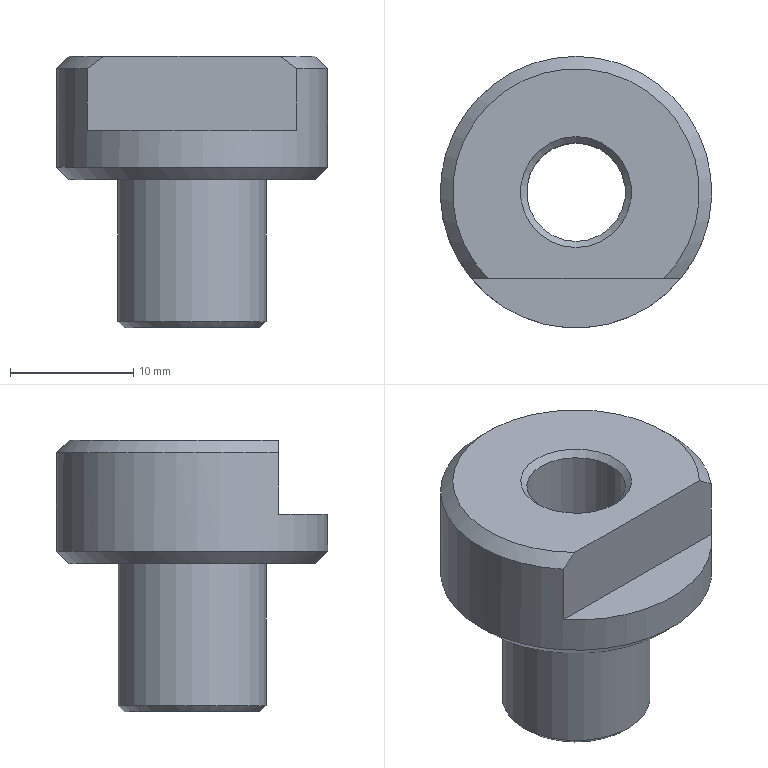Component | NX | DRILL_BUSH | 1 solid | 13 faces | box 22 x 22 x 22 mm | volume 3700 mm3 | plane 5 | cone 5 | cylinder 3 | commonest cylinder face diameters 12 x1 22 x1 8 x1
STEP:
#1=CARTESIAN_POINT('',(0.,0.,0.));
#2=DIRECTION('',(0.,0.,1.));
#3=DIRECTION('',(1.,0.,0.));
#4=AXIS2_PLACEMENT_3D('',#1,#2,#3);
#5=CARTESIAN_POINT('',(-15.,-13.5,92.));
#6=VERTEX_POINT('',#5);
#7=CARTESIAN_POINT('',(-15.,-18.,92.));
#8=DIRECTION('',(0.,0.,1.));
#9=DIRECTION('',(0.,1.,0.));
#10=AXIS2_PLACEMENT_3D('',#7,#8,#9);
#11=CIRCLE('',#10,4.5);
#12=CARTESIAN_POINT('',(-15.,-18.,92.));
#13=DIRECTION('',(0.,0.,-1.));
#14=DIRECTION('',(0.,1.,0.));
#15=AXIS2_PLACEMENT_3D('',#12,#13,#14);
#16=PLANE('',#15);
#17=CARTESIAN_POINT('',(4.5,0.));
#18=CARTESIAN_POINT('',(4.5,-7.794));
#19=CARTESIAN_POINT('',(-2.25,-3.897));
#20=CARTESIAN_POINT('',(-9.,-0.));
#21=CARTESIAN_POINT('',(-2.25,3.897));
#22=CARTESIAN_POINT('',(4.5,7.794));
#23=CARTESIAN_POINT('',(4.5,0.));
#24=(BOUNDED_CURVE()B_SPLINE_CURVE(2,(#17,#18,#19,#20,#21,#22,#23),.UNSPECIFIED.,.T.,.F.)B_SPLINE_CURVE_WITH_KNOTS((1,2,2,2,2,1),(-2.094,0.,2.094,4.189,6.283,8.378),.UNSPECIFIED.)CURVE()GEOMETRIC_REPRESENTATION_ITEM()RATIONAL_B_SPLINE_CURVE((1.,0.5,1.,0.5,1.,0.5,1.))REPRESENTATION_ITEM(''));
#25=(GEOMETRIC_REPRESENTATION_CONTEXT(2)PARAMETRIC_REPRESENTATION_CONTEXT()REPRESENTATION_CONTEXT('',''));
#26=DEFINITIONAL_REPRESENTATION('',(#24),#25);
#27=PCURVE('',#16,#26);
#28=CARTESIAN_POINT('',(-15.,-18.,92.5));
#29=DIRECTION('',(0.,0.,-1.));
#30=DIRECTION('',(0.,1.,0.));
#31=AXIS2_PLACEMENT_3D('',#28,#29,#30);
#32=CONICAL_SURFACE('',#31,4.,0.7854);
#33=CARTESIAN_POINT('',(6.283,0.5));
#34=DIRECTION('',(-1.,0.));
#35=VECTOR('',#34,1.);
#36=LINE('',#33,#35);
#37=(GEOMETRIC_REPRESENTATION_CONTEXT(2)PARAMETRIC_REPRESENTATION_CONTEXT()REPRESENTATION_CONTEXT('',''));
#38=DEFINITIONAL_REPRESENTATION('',(#36),#37);
#39=PCURVE('',#32,#38);
#40=SURFACE_CURVE('',#11,(#27,#39),.PCURVE_S1.);
#41=EDGE_CURVE('',#6,#6,#40,.T.);
#42=ORIENTED_EDGE('',*,*,#41,.T.);
#43=EDGE_LOOP('',(#42));
#44=FACE_BOUND('',#43,.T.);
#45=CARTESIAN_POINT('',(-15.,-12.5,92.));
#46=VERTEX_POINT('',#45);
#47=CARTESIAN_POINT('',(-15.,-18.,92.));
#48=DIRECTION('',(0.,0.,-1.));
#49=DIRECTION('',(0.,1.,0.));
#50=AXIS2_PLACEMENT_3D('',#47,#48,#49);
#51=CIRCLE('',#50,5.5);
#52=CARTESIAN_POINT('',(0.,0.));
#53=DIRECTION('',(1.,0.));
#54=AXIS2_PLACEMENT_2D('',#52,#53);
#55=CIRCLE('',#54,5.5);
#56=(GEOMETRIC_REPRESENTATION_CONTEXT(2)PARAMETRIC_REPRESENTATION_CONTEXT()REPRESENTATION_CONTEXT('',''));
#57=DEFINITIONAL_REPRESENTATION('',(#55),#56);
#58=PCURVE('',#16,#57);
#59=CARTESIAN_POINT('',(-15.,-18.,92.5));
#60=DIRECTION('',(0.,0.,1.));
#61=DIRECTION('',(0.,-1.,0.));
#62=AXIS2_PLACEMENT_3D('',#59,#60,#61);
#63=CONICAL_SURFACE('',#62,6.,0.7854);
#64=CARTESIAN_POINT('',(9.425,-0.5));
#65=DIRECTION('',(-1.,0.));
#66=VECTOR('',#65,1.);
#67=LINE('',#64,#66);
#68=(GEOMETRIC_REPRESENTATION_CONTEXT(2)PARAMETRIC_REPRESENTATION_CONTEXT()REPRESENTATION_CONTEXT('',''));
#69=DEFINITIONAL_REPRESENTATION('',(#67),#68);
#70=PCURVE('',#63,#69);
#71=SURFACE_CURVE('',#51,(#58,#70),.PCURVE_S1.);
#72=EDGE_CURVE('',#46,#46,#71,.T.);
#73=ORIENTED_EDGE('',*,*,#72,.T.);
#74=EDGE_LOOP('',(#73));
#75=FACE_BOUND('',#74,.T.);
#76=ADVANCED_FACE('',(#44,#75),#16,.T.);
#77=CARTESIAN_POINT('',(-15.,-12.,92.5));
#78=VERTEX_POINT('',#77);
#79=CARTESIAN_POINT('',(-15.,-18.,92.5));
#80=DIRECTION('',(0.,0.,1.));
#81=DIRECTION('',(0.,1.,0.));
#82=AXIS2_PLACEMENT_3D('',#79,#80,#81);
#83=CIRCLE('',#82,6.);
#84=CARTESIAN_POINT('',(-15.,-18.,92.));
#85=DIRECTION('',(0.,0.,1.));
#86=DIRECTION('',(0.,-1.,0.));
#87=AXIS2_PLACEMENT_3D('',#84,#85,#86);
#88=CYLINDRICAL_SURFACE('',#87,6.);
#89=CARTESIAN_POINT('',(3.142,0.5));
#90=DIRECTION('',(1.,0.));
#91=VECTOR('',#90,1.);
#92=LINE('',#89,#91);
#93=(GEOMETRIC_REPRESENTATION_CONTEXT(2)PARAMETRIC_REPRESENTATION_CONTEXT()REPRESENTATION_CONTEXT('',''));
#94=DEFINITIONAL_REPRESENTATION('',(#92),#93);
#95=PCURVE('',#88,#94);
#96=CARTESIAN_POINT('',(3.142,0.));
#97=DIRECTION('',(1.,0.));
#98=VECTOR('',#97,1.);
#99=LINE('',#96,#98);
#100=(GEOMETRIC_REPRESENTATION_CONTEXT(2)PARAMETRIC_REPRESENTATION_CONTEXT()REPRESENTATION_CONTEXT('',''));
#101=DEFINITIONAL_REPRESENTATION('',(#99),#100);
#102=PCURVE('',#63,#101);
#103=SURFACE_CURVE('',#83,(#95,#102),.PCURVE_S1.);
#104=EDGE_CURVE('',#78,#78,#103,.T.);
#105=ORIENTED_EDGE('',*,*,#104,.T.);
#106=CARTESIAN_POINT('',(-15.,-12.,104.));
#107=VERTEX_POINT('',#106);
#108=CARTESIAN_POINT('',(-15.,-12.,92.5));
#109=CARTESIAN_POINT('',(-15.,-12.,104.));
#110=B_SPLINE_CURVE_WITH_KNOTS('',1,(#108,#109),.UNSPECIFIED.,.F.,.F.,(2,2),(0.5,12.),.PIECEWISE_BEZIER_KNOTS.);
#111=CARTESIAN_POINT('',(9.425,0.));
#112=DIRECTION('',(0.,1.));
#113=VECTOR('',#112,1.);
#114=LINE('',#111,#113);
#115=(GEOMETRIC_REPRESENTATION_CONTEXT(2)PARAMETRIC_REPRESENTATION_CONTEXT()REPRESENTATION_CONTEXT('',''));
#116=DEFINITIONAL_REPRESENTATION('',(#114),#115);
#117=PCURVE('',#88,#116);
#118=CARTESIAN_POINT('',(3.142,0.));
#119=DIRECTION('',(0.,1.));
#120=VECTOR('',#119,1.);
#121=LINE('',#118,#120);
#122=(GEOMETRIC_REPRESENTATION_CONTEXT(2)PARAMETRIC_REPRESENTATION_CONTEXT()REPRESENTATION_CONTEXT('',''));
#123=DEFINITIONAL_REPRESENTATION('',(#121),#122);
#124=PCURVE('',#88,#123);
#125=SEAM_CURVE('',#110,(#117,#124),.PCURVE_S1.);
#126=EDGE_CURVE('',#78,#107,#125,.T.);
#127=ORIENTED_EDGE('',*,*,#126,.T.);
#128=CARTESIAN_POINT('',(-15.,-18.,104.));
#129=DIRECTION('',(0.,0.,1.));
#130=DIRECTION('',(0.,1.,0.));
#131=AXIS2_PLACEMENT_3D('',#128,#129,#130);
#132=CIRCLE('',#131,6.);
#133=CARTESIAN_POINT('',(3.142,12.));
#134=DIRECTION('',(1.,0.));
#135=VECTOR('',#134,1.);
#136=LINE('',#133,#135);
#137=(GEOMETRIC_REPRESENTATION_CONTEXT(2)PARAMETRIC_REPRESENTATION_CONTEXT()REPRESENTATION_CONTEXT('',''));
#138=DEFINITIONAL_REPRESENTATION('',(#136),#137);
#139=PCURVE('',#88,#138);
#140=CARTESIAN_POINT('',(-15.,-18.,104.));
#141=DIRECTION('',(0.,0.,-1.));
#142=DIRECTION('',(0.,1.,0.));
#143=AXIS2_PLACEMENT_3D('',#140,#141,#142);
#144=PLANE('',#143);
#145=CARTESIAN_POINT('',(6.,0.));
#146=CARTESIAN_POINT('',(6.,-10.392));
#147=CARTESIAN_POINT('',(-3.,-5.196));
#148=CARTESIAN_POINT('',(-12.,-0.));
#149=CARTESIAN_POINT('',(-3.,5.196));
#150=CARTESIAN_POINT('',(6.,10.392));
#151=CARTESIAN_POINT('',(6.,0.));
#152=(BOUNDED_CURVE()B_SPLINE_CURVE(2,(#145,#146,#147,#148,#149,#150,#151),.UNSPECIFIED.,.T.,.F.)B_SPLINE_CURVE_WITH_KNOTS((1,2,2,2,2,1),(-2.094,0.,2.094,4.189,6.283,8.378),.UNSPECIFIED.)CURVE()GEOMETRIC_REPRESENTATION_ITEM()RATIONAL_B_SPLINE_CURVE((1.,0.5,1.,0.5,1.,0.5,1.))REPRESENTATION_ITEM(''));
#153=(GEOMETRIC_REPRESENTATION_CONTEXT(2)PARAMETRIC_REPRESENTATION_CONTEXT()REPRESENTATION_CONTEXT('',''));
#154=DEFINITIONAL_REPRESENTATION('',(#152),#153);
#155=PCURVE('',#144,#154);
#156=SURFACE_CURVE('',#132,(#139,#155),.PCURVE_S1.);
#157=EDGE_CURVE('',#107,#107,#156,.T.);
#158=ORIENTED_EDGE('',*,*,#157,.F.);
#159=ORIENTED_EDGE('',*,*,#126,.F.);
#160=EDGE_LOOP('',(#105,#127,#158,#159));
#161=FACE_BOUND('',#160,.T.);
#162=ADVANCED_FACE('',(#161),#88,.T.);
#163=CARTESIAN_POINT('',(-15.,-22.5,114.));
#164=VERTEX_POINT('',#163);
#165=CARTESIAN_POINT('',(-15.,-18.,114.));
#166=DIRECTION('',(0.,0.,-1.));
#167=DIRECTION('',(0.,-1.,0.));
#168=AXIS2_PLACEMENT_3D('',#165,#166,#167);
#169=CIRCLE('',#168,4.5);
#170=CARTESIAN_POINT('',(-15.,-18.,114.));
#171=DIRECTION('',(0.,0.,1.));
#172=DIRECTION('',(0.,-1.,0.));
#173=AXIS2_PLACEMENT_3D('',#170,#171,#172);
#174=PLANE('',#173);
#175=CARTESIAN_POINT('',(4.5,0.));
#176=CARTESIAN_POINT('',(4.5,-7.794));
#177=CARTESIAN_POINT('',(-2.25,-3.897));
#178=CARTESIAN_POINT('',(-9.,-0.));
#179=CARTESIAN_POINT('',(-2.25,3.897));
#180=CARTESIAN_POINT('',(4.5,7.794));
#181=CARTESIAN_POINT('',(4.5,0.));
#182=(BOUNDED_CURVE()B_SPLINE_CURVE(2,(#175,#176,#177,#178,#179,#180,#181),.UNSPECIFIED.,.T.,.F.)B_SPLINE_CURVE_WITH_KNOTS((1,2,2,2,2,1),(-2.094,0.,2.094,4.189,6.283,8.378),.UNSPECIFIED.)CURVE()GEOMETRIC_REPRESENTATION_ITEM()RATIONAL_B_SPLINE_CURVE((1.,0.5,1.,0.5,1.,0.5,1.))REPRESENTATION_ITEM(''));
#183=(GEOMETRIC_REPRESENTATION_CONTEXT(2)PARAMETRIC_REPRESENTATION_CONTEXT()REPRESENTATION_CONTEXT('',''));
#184=DEFINITIONAL_REPRESENTATION('',(#182),#183);
#185=PCURVE('',#174,#184);
#186=CARTESIAN_POINT('',(-15.,-18.,114.));
#187=DIRECTION('',(0.,0.,1.));
#188=DIRECTION('',(0.,-1.,0.));
#189=AXIS2_PLACEMENT_3D('',#186,#187,#188);
#190=CONICAL_SURFACE('',#189,4.5,0.7854);
#191=CARTESIAN_POINT('',(6.283,0.));
#192=DIRECTION('',(-1.,0.));
#193=VECTOR('',#192,1.);
#194=LINE('',#191,#193);
#195=(GEOMETRIC_REPRESENTATION_CONTEXT(2)PARAMETRIC_REPRESENTATION_CONTEXT()REPRESENTATION_CONTEXT('',''));
#196=DEFINITIONAL_REPRESENTATION('',(#194),#195);
#197=PCURVE('',#190,#196);
#198=SURFACE_CURVE('',#169,(#185,#197),.PCURVE_S1.);
#199=EDGE_CURVE('',#164,#164,#198,.T.);
#200=ORIENTED_EDGE('',*,*,#199,.T.);
#201=EDGE_LOOP('',(#200));
#202=FACE_BOUND('',#201,.T.);
#203=CARTESIAN_POINT('',(-7.859,-25.,114.));
#204=VERTEX_POINT('',#203);
#205=CARTESIAN_POINT('',(-22.141,-25.,114.));
#206=VERTEX_POINT('',#205);
#207=CARTESIAN_POINT('',(-2.,-25.,114.));
#208=DIRECTION('',(-1.,-0.,0.));
#209=VECTOR('',#208,1.);
#210=LINE('',#207,#209);
#211=CARTESIAN_POINT('',(7.,13.));
#212=DIRECTION('',(0.,-1.));
#213=VECTOR('',#212,1.);
#214=LINE('',#211,#213);
#215=(GEOMETRIC_REPRESENTATION_CONTEXT(2)PARAMETRIC_REPRESENTATION_CONTEXT()REPRESENTATION_CONTEXT('',''));
#216=DEFINITIONAL_REPRESENTATION('',(#214),#215);
#217=PCURVE('',#174,#216);
#218=CARTESIAN_POINT('',(-2.,-25.,108.));
#219=DIRECTION('',(-0.,1.,0.));
#220=DIRECTION('',(-1.,-0.,0.));
#221=AXIS2_PLACEMENT_3D('',#218,#219,#220);
#222=PLANE('',#221);
#223=CARTESIAN_POINT('',(0.,6.));
#224=DIRECTION('',(1.,0.));
#225=VECTOR('',#224,1.);
#226=LINE('',#223,#225);
#227=(GEOMETRIC_REPRESENTATION_CONTEXT(2)PARAMETRIC_REPRESENTATION_CONTEXT()REPRESENTATION_CONTEXT('',''));
#228=DEFINITIONAL_REPRESENTATION('',(#226),#227);
#229=PCURVE('',#222,#228);
#230=SURFACE_CURVE('',#210,(#217,#229),.PCURVE_S1.);
#231=EDGE_CURVE('',#204,#206,#230,.T.);
#232=ORIENTED_EDGE('',*,*,#231,.F.);
#233=CARTESIAN_POINT('',(-15.,-18.,114.));
#234=DIRECTION('',(0.,0.,1.));
#235=DIRECTION('',(0.,-1.,0.));
#236=AXIS2_PLACEMENT_3D('',#233,#234,#235);
#237=CIRCLE('',#236,10.);
#238=CARTESIAN_POINT('',(0.,0.));
#239=DIRECTION('',(1.,0.));
#240=AXIS2_PLACEMENT_2D('',#238,#239);
#241=CIRCLE('',#240,10.);
#242=(GEOMETRIC_REPRESENTATION_CONTEXT(2)PARAMETRIC_REPRESENTATION_CONTEXT()REPRESENTATION_CONTEXT('',''));
#243=DEFINITIONAL_REPRESENTATION('',(#241),#242);
#244=PCURVE('',#174,#243);
#245=CARTESIAN_POINT('',(-15.,-18.,113.));
#246=DIRECTION('',(0.,0.,-1.));
#247=DIRECTION('',(0.,1.,0.));
#248=AXIS2_PLACEMENT_3D('',#245,#246,#247);
#249=CONICAL_SURFACE('',#248,11.,0.7854);
#250=CARTESIAN_POINT('',(3.142,-1.));
#251=DIRECTION('',(-1.,0.));
#252=VECTOR('',#251,1.);
#253=LINE('',#250,#252);
#254=(GEOMETRIC_REPRESENTATION_CONTEXT(2)PARAMETRIC_REPRESENTATION_CONTEXT()REPRESENTATION_CONTEXT('',''));
#255=DEFINITIONAL_REPRESENTATION('',(#253),#254);
#256=PCURVE('',#249,#255);
#257=SURFACE_CURVE('',#237,(#244,#256),.PCURVE_S1.);
#258=EDGE_CURVE('',#204,#206,#257,.T.);
#259=ORIENTED_EDGE('',*,*,#258,.T.);
#260=EDGE_LOOP('',(#232,#259));
#261=FACE_BOUND('',#260,.T.);
#262=ADVANCED_FACE('',(#202,#261),#174,.T.);
#263=CARTESIAN_POINT('',(-15.,-8.,104.));
#264=VERTEX_POINT('',#263);
#265=CARTESIAN_POINT('',(-15.,-18.,104.));
#266=DIRECTION('',(0.,0.,-1.));
#267=DIRECTION('',(0.,1.,0.));
#268=AXIS2_PLACEMENT_3D('',#265,#266,#267);
#269=CIRCLE('',#268,10.);
#270=CARTESIAN_POINT('',(0.,0.));
#271=DIRECTION('',(1.,0.));
#272=AXIS2_PLACEMENT_2D('',#270,#271);
#273=CIRCLE('',#272,10.);
#274=(GEOMETRIC_REPRESENTATION_CONTEXT(2)PARAMETRIC_REPRESENTATION_CONTEXT()REPRESENTATION_CONTEXT('',''));
#275=DEFINITIONAL_REPRESENTATION('',(#273),#274);
#276=PCURVE('',#144,#275);
#277=CARTESIAN_POINT('',(-15.,-18.,105.));
#278=DIRECTION('',(0.,0.,1.));
#279=DIRECTION('',(0.,-1.,0.));
#280=AXIS2_PLACEMENT_3D('',#277,#278,#279);
#281=CONICAL_SURFACE('',#280,11.,0.7854);
#282=CARTESIAN_POINT('',(9.425,-1.));
#283=DIRECTION('',(-1.,0.));
#284=VECTOR('',#283,1.);
#285=LINE('',#282,#284);
#286=(GEOMETRIC_REPRESENTATION_CONTEXT(2)PARAMETRIC_REPRESENTATION_CONTEXT()REPRESENTATION_CONTEXT('',''));
#287=DEFINITIONAL_REPRESENTATION('',(#285),#286);
#288=PCURVE('',#281,#287);
#289=SURFACE_CURVE('',#269,(#276,#288),.PCURVE_S1.);
#290=EDGE_CURVE('',#264,#264,#289,.T.);
#291=ORIENTED_EDGE('',*,*,#290,.T.);
#292=EDGE_LOOP('',(#291));
#293=FACE_BOUND('',#292,.T.);
#294=ORIENTED_EDGE('',*,*,#157,.T.);
#295=EDGE_LOOP('',(#294));
#296=FACE_BOUND('',#295,.T.);
#297=ADVANCED_FACE('',(#293,#296),#144,.T.);
#298=CARTESIAN_POINT('',(-15.,-7.,105.));
#299=VERTEX_POINT('',#298);
#300=CARTESIAN_POINT('',(-6.515,-25.,105.));
#301=VERTEX_POINT('',#300);
#302=CARTESIAN_POINT('',(-15.,-18.,105.));
#303=DIRECTION('',(0.,0.,1.));
#304=DIRECTION('',(0.,1.,0.));
#305=AXIS2_PLACEMENT_3D('',#302,#303,#304);
#306=CIRCLE('',#305,11.);
#307=CARTESIAN_POINT('',(-15.,-18.,104.));
#308=DIRECTION('',(0.,0.,1.));
#309=DIRECTION('',(0.,-1.,0.));
#310=AXIS2_PLACEMENT_3D('',#307,#308,#309);
#311=CYLINDRICAL_SURFACE('',#310,11.);
#312=CARTESIAN_POINT('',(3.142,1.));
#313=DIRECTION('',(1.,0.));
#314=VECTOR('',#313,1.);
#315=LINE('',#312,#314);
#316=(GEOMETRIC_REPRESENTATION_CONTEXT(2)PARAMETRIC_REPRESENTATION_CONTEXT()REPRESENTATION_CONTEXT('',''));
#317=DEFINITIONAL_REPRESENTATION('',(#315),#316);
#318=PCURVE('',#311,#317);
#319=CARTESIAN_POINT('',(3.142,0.));
#320=DIRECTION('',(1.,0.));
#321=VECTOR('',#320,1.);
#322=LINE('',#319,#321);
#323=(GEOMETRIC_REPRESENTATION_CONTEXT(2)PARAMETRIC_REPRESENTATION_CONTEXT()REPRESENTATION_CONTEXT('',''));
#324=DEFINITIONAL_REPRESENTATION('',(#322),#323);
#325=PCURVE('',#281,#324);
#326=SURFACE_CURVE('',#306,(#318,#325),.PCURVE_S1.);
#327=EDGE_CURVE('',#299,#301,#326,.T.);
#328=ORIENTED_EDGE('',*,*,#327,.T.);
#329=CARTESIAN_POINT('',(-6.515,-25.,108.));
#330=VERTEX_POINT('',#329);
#331=CARTESIAN_POINT('',(-6.515,-25.,105.));
#332=CARTESIAN_POINT('',(-6.515,-25.,108.));
#333=B_SPLINE_CURVE_WITH_KNOTS('',1,(#331,#332),.UNSPECIFIED.,.F.,.F.,(2,2),(1.,4.),.PIECEWISE_BEZIER_KNOTS.);
#334=CARTESIAN_POINT('',(7.164,0.));
#335=DIRECTION('',(0.,1.));
#336=VECTOR('',#335,1.);
#337=LINE('',#334,#336);
#338=(GEOMETRIC_REPRESENTATION_CONTEXT(2)PARAMETRIC_REPRESENTATION_CONTEXT()REPRESENTATION_CONTEXT('',''));
#339=DEFINITIONAL_REPRESENTATION('',(#337),#338);
#340=PCURVE('',#311,#339);
#341=CARTESIAN_POINT('',(0.881,0.));
#342=DIRECTION('',(0.,1.));
#343=VECTOR('',#342,1.);
#344=LINE('',#341,#343);
#345=(GEOMETRIC_REPRESENTATION_CONTEXT(2)PARAMETRIC_REPRESENTATION_CONTEXT()REPRESENTATION_CONTEXT('',''));
#346=DEFINITIONAL_REPRESENTATION('',(#344),#345);
#347=PCURVE('',#311,#346);
#348=SEAM_CURVE('',#333,(#340,#347),.PCURVE_S1.);
#349=EDGE_CURVE('',#301,#330,#348,.T.);
#350=ORIENTED_EDGE('',*,*,#349,.T.);
#351=CARTESIAN_POINT('',(-23.485,-25.,108.));
#352=VERTEX_POINT('',#351);
#353=CARTESIAN_POINT('',(-15.,-18.,108.));
#354=DIRECTION('',(0.,0.,-1.));
#355=DIRECTION('',(0.,-1.,0.));
#356=AXIS2_PLACEMENT_3D('',#353,#354,#355);
#357=CIRCLE('',#356,11.);
#358=CARTESIAN_POINT('',(12.566,4.));
#359=DIRECTION('',(-1.,0.));
#360=VECTOR('',#359,1.);
#361=LINE('',#358,#360);
#362=(GEOMETRIC_REPRESENTATION_CONTEXT(2)PARAMETRIC_REPRESENTATION_CONTEXT()REPRESENTATION_CONTEXT('',''));
#363=DEFINITIONAL_REPRESENTATION('',(#361),#362);
#364=PCURVE('',#311,#363);
#365=CARTESIAN_POINT('',(-15.,-18.,108.));
#366=DIRECTION('',(0.,0.,1.));
#367=DIRECTION('',(0.,-1.,0.));
#368=AXIS2_PLACEMENT_3D('',#365,#366,#367);
#369=PLANE('',#368);
#370=CARTESIAN_POINT('',(11.,0.));
#371=CARTESIAN_POINT('',(11.,-19.053));
#372=CARTESIAN_POINT('',(-5.5,-9.526));
#373=CARTESIAN_POINT('',(-22.,-0.));
#374=CARTESIAN_POINT('',(-5.5,9.526));
#375=CARTESIAN_POINT('',(11.,19.053));
#376=CARTESIAN_POINT('',(11.,0.));
#377=(BOUNDED_CURVE()B_SPLINE_CURVE(2,(#370,#371,#372,#373,#374,#375,#376),.UNSPECIFIED.,.T.,.F.)B_SPLINE_CURVE_WITH_KNOTS((1,2,2,2,2,1),(-2.094,0.,2.094,4.189,6.283,8.378),.UNSPECIFIED.)CURVE()GEOMETRIC_REPRESENTATION_ITEM()RATIONAL_B_SPLINE_CURVE((1.,0.5,1.,0.5,1.,0.5,1.))REPRESENTATION_ITEM(''));
#378=(GEOMETRIC_REPRESENTATION_CONTEXT(2)PARAMETRIC_REPRESENTATION_CONTEXT()REPRESENTATION_CONTEXT('',''));
#379=DEFINITIONAL_REPRESENTATION('',(#377),#378);
#380=PCURVE('',#369,#379);
#381=SURFACE_CURVE('',#357,(#364,#380),.PCURVE_S1.);
#382=EDGE_CURVE('',#330,#352,#381,.T.);
#383=ORIENTED_EDGE('',*,*,#382,.T.);
#384=CARTESIAN_POINT('',(-23.485,-25.,113.));
#385=VERTEX_POINT('',#384);
#386=CARTESIAN_POINT('',(-23.485,-25.,104.));
#387=DIRECTION('',(0.,0.,-1.));
#388=VECTOR('',#387,1.);
#389=LINE('',#386,#388);
#390=CARTESIAN_POINT('',(5.402,0.));
#391=DIRECTION('',(0.,-1.));
#392=VECTOR('',#391,1.);
#393=LINE('',#390,#392);
#394=(GEOMETRIC_REPRESENTATION_CONTEXT(2)PARAMETRIC_REPRESENTATION_CONTEXT()REPRESENTATION_CONTEXT('',''));
#395=DEFINITIONAL_REPRESENTATION('',(#393),#394);
#396=PCURVE('',#311,#395);
#397=CARTESIAN_POINT('',(21.485,-4.));
#398=DIRECTION('',(0.,-1.));
#399=VECTOR('',#398,1.);
#400=LINE('',#397,#399);
#401=(GEOMETRIC_REPRESENTATION_CONTEXT(2)PARAMETRIC_REPRESENTATION_CONTEXT()REPRESENTATION_CONTEXT('',''));
#402=DEFINITIONAL_REPRESENTATION('',(#400),#401);
#403=PCURVE('',#222,#402);
#404=SURFACE_CURVE('',#389,(#396,#403),.PCURVE_S1.);
#405=EDGE_CURVE('',#385,#352,#404,.T.);
#406=ORIENTED_EDGE('',*,*,#405,.F.);
#407=CARTESIAN_POINT('',(-6.515,-25.,113.));
#408=VERTEX_POINT('',#407);
#409=CARTESIAN_POINT('',(-15.,-18.,113.));
#410=DIRECTION('',(0.,0.,-1.));
#411=DIRECTION('',(0.,-1.,0.));
#412=AXIS2_PLACEMENT_3D('',#409,#410,#411);
#413=CIRCLE('',#412,11.);
#414=CARTESIAN_POINT('',(6.283,9.));
#415=DIRECTION('',(-1.,0.));
#416=VECTOR('',#415,1.);
#417=LINE('',#414,#416);
#418=(GEOMETRIC_REPRESENTATION_CONTEXT(2)PARAMETRIC_REPRESENTATION_CONTEXT()REPRESENTATION_CONTEXT('',''));
#419=DEFINITIONAL_REPRESENTATION('',(#417),#418);
#420=PCURVE('',#311,#419);
#421=CARTESIAN_POINT('',(-3.142,0.));
#422=DIRECTION('',(1.,0.));
#423=VECTOR('',#422,1.);
#424=LINE('',#421,#423);
#425=(GEOMETRIC_REPRESENTATION_CONTEXT(2)PARAMETRIC_REPRESENTATION_CONTEXT()REPRESENTATION_CONTEXT('',''));
#426=DEFINITIONAL_REPRESENTATION('',(#424),#425);
#427=PCURVE('',#249,#426);
#428=SURFACE_CURVE('',#413,(#420,#427),.PCURVE_S1.);
#429=EDGE_CURVE('',#385,#408,#428,.T.);
#430=ORIENTED_EDGE('',*,*,#429,.T.);
#431=CARTESIAN_POINT('',(-6.515,-25.,104.));
#432=DIRECTION('',(0.,0.,1.));
#433=VECTOR('',#432,1.);
#434=LINE('',#431,#433);
#435=CARTESIAN_POINT('',(0.881,0.));
#436=DIRECTION('',(0.,1.));
#437=VECTOR('',#436,1.);
#438=LINE('',#435,#437);
#439=(GEOMETRIC_REPRESENTATION_CONTEXT(2)PARAMETRIC_REPRESENTATION_CONTEXT()REPRESENTATION_CONTEXT('',''));
#440=DEFINITIONAL_REPRESENTATION('',(#438),#439);
#441=PCURVE('',#311,#440);
#442=CARTESIAN_POINT('',(4.515,-4.));
#443=DIRECTION('',(0.,1.));
#444=VECTOR('',#443,1.);
#445=LINE('',#442,#444);
#446=(GEOMETRIC_REPRESENTATION_CONTEXT(2)PARAMETRIC_REPRESENTATION_CONTEXT()REPRESENTATION_CONTEXT('',''));
#447=DEFINITIONAL_REPRESENTATION('',(#445),#446);
#448=PCURVE('',#222,#447);
#449=SURFACE_CURVE('',#434,(#441,#448),.PCURVE_S1.);
#450=EDGE_CURVE('',#330,#408,#449,.T.);
#451=ORIENTED_EDGE('',*,*,#450,.F.);
#452=ORIENTED_EDGE('',*,*,#349,.F.);
#453=CARTESIAN_POINT('',(-15.,-18.,105.));
#454=DIRECTION('',(0.,0.,1.));
#455=DIRECTION('',(0.,1.,0.));
#456=AXIS2_PLACEMENT_3D('',#453,#454,#455);
#457=CIRCLE('',#456,11.);
#458=CARTESIAN_POINT('',(-3.142,1.));
#459=DIRECTION('',(1.,0.));
#460=VECTOR('',#459,1.);
#461=LINE('',#458,#460);
#462=(GEOMETRIC_REPRESENTATION_CONTEXT(2)PARAMETRIC_REPRESENTATION_CONTEXT()REPRESENTATION_CONTEXT('',''));
#463=DEFINITIONAL_REPRESENTATION('',(#461),#462);
#464=PCURVE('',#311,#463);
#465=CARTESIAN_POINT('',(3.142,0.));
#466=DIRECTION('',(1.,0.));
#467=VECTOR('',#466,1.);
#468=LINE('',#465,#467);
#469=(GEOMETRIC_REPRESENTATION_CONTEXT(2)PARAMETRIC_REPRESENTATION_CONTEXT()REPRESENTATION_CONTEXT('',''));
#470=DEFINITIONAL_REPRESENTATION('',(#468),#469);
#471=PCURVE('',#281,#470);
#472=SURFACE_CURVE('',#457,(#464,#471),.PCURVE_S1.);
#473=EDGE_CURVE('',#301,#299,#472,.T.);
#474=ORIENTED_EDGE('',*,*,#473,.T.);
#475=EDGE_LOOP('',(#328,#350,#383,#406,#430,#451,#452,#474));
#476=FACE_BOUND('',#475,.T.);
#477=ADVANCED_FACE('',(#476),#311,.T.);
#478=ORIENTED_EDGE('',*,*,#450,.T.);
#479=CARTESIAN_POINT('',(-6.515,-25.,113.));
#480=CARTESIAN_POINT('',(-6.957,-25.,113.341));
#481=CARTESIAN_POINT('',(-7.404,-25.,113.676));
#482=CARTESIAN_POINT('',(-7.859,-25.,114.));
#483=B_SPLINE_CURVE_WITH_KNOTS('',3,(#479,#480,#481,#482),.UNSPECIFIED.,.F.,.F.,(4,4),(0.,1.),.PIECEWISE_BEZIER_KNOTS.);
#484=CARTESIAN_POINT('',(4.515,5.));
#485=CARTESIAN_POINT('',(4.957,5.341));
#486=CARTESIAN_POINT('',(5.404,5.676));
#487=CARTESIAN_POINT('',(5.859,6.));
#488=B_SPLINE_CURVE_WITH_KNOTS('',3,(#484,#485,#486,#487),.UNSPECIFIED.,.F.,.F.,(4,4),(0.,1.),.PIECEWISE_BEZIER_KNOTS.);
#489=(GEOMETRIC_REPRESENTATION_CONTEXT(2)PARAMETRIC_REPRESENTATION_CONTEXT()REPRESENTATION_CONTEXT('',''));
#490=DEFINITIONAL_REPRESENTATION('',(#488),#489);
#491=PCURVE('',#222,#490);
#492=CARTESIAN_POINT('',(2.261,-0.));
#493=CARTESIAN_POINT('',(2.346,-1.));
#494=B_SPLINE_CURVE_WITH_KNOTS('',1,(#492,#493),.UNSPECIFIED.,.F.,.F.,(2,2),(0.,1.),.PIECEWISE_BEZIER_KNOTS.);
#495=(GEOMETRIC_REPRESENTATION_CONTEXT(2)PARAMETRIC_REPRESENTATION_CONTEXT()REPRESENTATION_CONTEXT('',''));
#496=DEFINITIONAL_REPRESENTATION('',(#494),#495);
#497=PCURVE('',#249,#496);
#498=SURFACE_CURVE('',#483,(#491,#497),.PCURVE_S1.);
#499=EDGE_CURVE('',#408,#204,#498,.T.);
#500=ORIENTED_EDGE('',*,*,#499,.T.);
#501=ORIENTED_EDGE('',*,*,#231,.T.);
#502=CARTESIAN_POINT('',(-22.141,-25.,114.));
#503=CARTESIAN_POINT('',(-22.596,-25.,113.676));
#504=CARTESIAN_POINT('',(-23.043,-25.,113.341));
#505=CARTESIAN_POINT('',(-23.485,-25.,113.));
#506=B_SPLINE_CURVE_WITH_KNOTS('',3,(#502,#503,#504,#505),.UNSPECIFIED.,.F.,.F.,(4,4),(0.,1.),.PIECEWISE_BEZIER_KNOTS.);
#507=CARTESIAN_POINT('',(20.141,6.));
#508=CARTESIAN_POINT('',(20.596,5.676));
#509=CARTESIAN_POINT('',(21.043,5.341));
#510=CARTESIAN_POINT('',(21.485,5.));
#511=B_SPLINE_CURVE_WITH_KNOTS('',3,(#507,#508,#509,#510),.UNSPECIFIED.,.F.,.F.,(4,4),(0.,1.),.PIECEWISE_BEZIER_KNOTS.);
#512=(GEOMETRIC_REPRESENTATION_CONTEXT(2)PARAMETRIC_REPRESENTATION_CONTEXT()REPRESENTATION_CONTEXT('',''));
#513=DEFINITIONAL_REPRESENTATION('',(#511),#512);
#514=PCURVE('',#222,#513);
#515=CARTESIAN_POINT('',(-2.346,-1.));
#516=CARTESIAN_POINT('',(-2.261,0.));
#517=B_SPLINE_CURVE_WITH_KNOTS('',1,(#515,#516),.UNSPECIFIED.,.F.,.F.,(2,2),(0.,1.),.PIECEWISE_BEZIER_KNOTS.);
#518=(GEOMETRIC_REPRESENTATION_CONTEXT(2)PARAMETRIC_REPRESENTATION_CONTEXT()REPRESENTATION_CONTEXT('',''));
#519=DEFINITIONAL_REPRESENTATION('',(#517),#518);
#520=PCURVE('',#249,#519);
#521=SURFACE_CURVE('',#506,(#514,#520),.PCURVE_S1.);
#522=EDGE_CURVE('',#206,#385,#521,.T.);
#523=ORIENTED_EDGE('',*,*,#522,.T.);
#524=ORIENTED_EDGE('',*,*,#405,.T.);
#525=CARTESIAN_POINT('',(-2.,-25.,108.));
#526=DIRECTION('',(1.,0.,0.));
#527=VECTOR('',#526,1.);
#528=LINE('',#525,#527);
#529=CARTESIAN_POINT('',(0.,0.));
#530=DIRECTION('',(-1.,0.));
#531=VECTOR('',#530,1.);
#532=LINE('',#529,#531);
#533=(GEOMETRIC_REPRESENTATION_CONTEXT(2)PARAMETRIC_REPRESENTATION_CONTEXT()REPRESENTATION_CONTEXT('',''));
#534=DEFINITIONAL_REPRESENTATION('',(#532),#533);
#535=PCURVE('',#222,#534);
#536=CARTESIAN_POINT('',(7.,13.));
#537=DIRECTION('',(-0.,1.));
#538=VECTOR('',#537,1.);
#539=LINE('',#536,#538);
#540=(GEOMETRIC_REPRESENTATION_CONTEXT(2)PARAMETRIC_REPRESENTATION_CONTEXT()REPRESENTATION_CONTEXT('',''));
#541=DEFINITIONAL_REPRESENTATION('',(#539),#540);
#542=PCURVE('',#369,#541);
#543=SURFACE_CURVE('',#528,(#535,#542),.PCURVE_S1.);
#544=EDGE_CURVE('',#352,#330,#543,.T.);
#545=ORIENTED_EDGE('',*,*,#544,.T.);
#546=EDGE_LOOP('',(#478,#500,#501,#523,#524,#545));
#547=FACE_BOUND('',#546,.T.);
#548=ADVANCED_FACE('',(#547),#222,.F.);
#549=ORIENTED_EDGE('',*,*,#544,.F.);
#550=ORIENTED_EDGE('',*,*,#382,.F.);
#551=EDGE_LOOP('',(#549,#550));
#552=FACE_BOUND('',#551,.T.);
#553=ADVANCED_FACE('',(#552),#369,.T.);
#554=CARTESIAN_POINT('',(-15.,-14.,92.5));
#555=VERTEX_POINT('',#554);
#556=CARTESIAN_POINT('',(-15.,-18.,92.5));
#557=DIRECTION('',(0.,0.,-1.));
#558=DIRECTION('',(0.,1.,0.));
#559=AXIS2_PLACEMENT_3D('',#556,#557,#558);
#560=CIRCLE('',#559,4.);
#561=CARTESIAN_POINT('',(-15.,-18.,114.));
#562=DIRECTION('',(0.,0.,-1.));
#563=DIRECTION('',(0.,1.,0.));
#564=AXIS2_PLACEMENT_3D('',#561,#562,#563);
#565=CYLINDRICAL_SURFACE('',#564,4.);
#566=CARTESIAN_POINT('',(0.,21.5));
#567=DIRECTION('',(1.,0.));
#568=VECTOR('',#567,1.);
#569=LINE('',#566,#568);
#570=(GEOMETRIC_REPRESENTATION_CONTEXT(2)PARAMETRIC_REPRESENTATION_CONTEXT()REPRESENTATION_CONTEXT('',''));
#571=DEFINITIONAL_REPRESENTATION('',(#569),#570);
#572=PCURVE('',#565,#571);
#573=CARTESIAN_POINT('',(0.,0.));
#574=DIRECTION('',(1.,0.));
#575=VECTOR('',#574,1.);
#576=LINE('',#573,#575);
#577=(GEOMETRIC_REPRESENTATION_CONTEXT(2)PARAMETRIC_REPRESENTATION_CONTEXT()REPRESENTATION_CONTEXT('',''));
#578=DEFINITIONAL_REPRESENTATION('',(#576),#577);
#579=PCURVE('',#32,#578);
#580=SURFACE_CURVE('',#560,(#572,#579),.PCURVE_S1.);
#581=EDGE_CURVE('',#555,#555,#580,.T.);
#582=ORIENTED_EDGE('',*,*,#581,.F.);
#583=CARTESIAN_POINT('',(-15.,-14.,113.5));
#584=VERTEX_POINT('',#583);
#585=CARTESIAN_POINT('',(-15.,-14.,113.5));
#586=CARTESIAN_POINT('',(-15.,-14.,92.5));
#587=B_SPLINE_CURVE_WITH_KNOTS('',1,(#585,#586),.UNSPECIFIED.,.F.,.F.,(2,2),(0.5,21.5),.PIECEWISE_BEZIER_KNOTS.);
#588=CARTESIAN_POINT('',(0.,0.));
#589=DIRECTION('',(0.,1.));
#590=VECTOR('',#589,1.);
#591=LINE('',#588,#590);
#592=(GEOMETRIC_REPRESENTATION_CONTEXT(2)PARAMETRIC_REPRESENTATION_CONTEXT()REPRESENTATION_CONTEXT('',''));
#593=DEFINITIONAL_REPRESENTATION('',(#591),#592);
#594=PCURVE('',#565,#593);
#595=CARTESIAN_POINT('',(6.283,0.));
#596=DIRECTION('',(0.,1.));
#597=VECTOR('',#596,1.);
#598=LINE('',#595,#597);
#599=(GEOMETRIC_REPRESENTATION_CONTEXT(2)PARAMETRIC_REPRESENTATION_CONTEXT()REPRESENTATION_CONTEXT('',''));
#600=DEFINITIONAL_REPRESENTATION('',(#598),#599);
#601=PCURVE('',#565,#600);
#602=SEAM_CURVE('',#587,(#594,#601),.PCURVE_S1.);
#603=EDGE_CURVE('',#584,#555,#602,.T.);
#604=ORIENTED_EDGE('',*,*,#603,.F.);
#605=CARTESIAN_POINT('',(-15.,-22.,113.5));
#606=VERTEX_POINT('',#605);
#607=CARTESIAN_POINT('',(-15.,-18.,113.5));
#608=DIRECTION('',(0.,0.,1.));
#609=DIRECTION('',(0.,-1.,0.));
#610=AXIS2_PLACEMENT_3D('',#607,#608,#609);
#611=CIRCLE('',#610,4.);
#612=CARTESIAN_POINT('',(3.142,0.5));
#613=DIRECTION('',(-1.,0.));
#614=VECTOR('',#613,1.);
#615=LINE('',#612,#614);
#616=(GEOMETRIC_REPRESENTATION_CONTEXT(2)PARAMETRIC_REPRESENTATION_CONTEXT()REPRESENTATION_CONTEXT('',''));
#617=DEFINITIONAL_REPRESENTATION('',(#615),#616);
#618=PCURVE('',#565,#617);
#619=CARTESIAN_POINT('',(0.,-0.5));
#620=DIRECTION('',(1.,0.));
#621=VECTOR('',#620,1.);
#622=LINE('',#619,#621);
#623=(GEOMETRIC_REPRESENTATION_CONTEXT(2)PARAMETRIC_REPRESENTATION_CONTEXT()REPRESENTATION_CONTEXT('',''));
#624=DEFINITIONAL_REPRESENTATION('',(#622),#623);
#625=PCURVE('',#190,#624);
#626=SURFACE_CURVE('',#611,(#618,#625),.PCURVE_S1.);
#627=EDGE_CURVE('',#606,#584,#626,.T.);
#628=ORIENTED_EDGE('',*,*,#627,.F.);
#629=CARTESIAN_POINT('',(-15.,-18.,113.5));
#630=DIRECTION('',(0.,0.,1.));
#631=DIRECTION('',(0.,-1.,0.));
#632=AXIS2_PLACEMENT_3D('',#629,#630,#631);
#633=CIRCLE('',#632,4.);
#634=CARTESIAN_POINT('',(9.425,0.5));
#635=DIRECTION('',(-1.,0.));
#636=VECTOR('',#635,1.);
#637=LINE('',#634,#636);
#638=(GEOMETRIC_REPRESENTATION_CONTEXT(2)PARAMETRIC_REPRESENTATION_CONTEXT()REPRESENTATION_CONTEXT('',''));
#639=DEFINITIONAL_REPRESENTATION('',(#637),#638);
#640=PCURVE('',#565,#639);
#641=CARTESIAN_POINT('',(0.,-0.5));
#642=DIRECTION('',(1.,0.));
#643=VECTOR('',#642,1.);
#644=LINE('',#641,#643);
#645=(GEOMETRIC_REPRESENTATION_CONTEXT(2)PARAMETRIC_REPRESENTATION_CONTEXT()REPRESENTATION_CONTEXT('',''));
#646=DEFINITIONAL_REPRESENTATION('',(#644),#645);
#647=PCURVE('',#190,#646);
#648=SURFACE_CURVE('',#633,(#640,#647),.PCURVE_S1.);
#649=EDGE_CURVE('',#584,#606,#648,.T.);
#650=ORIENTED_EDGE('',*,*,#649,.F.);
#651=ORIENTED_EDGE('',*,*,#603,.T.);
#652=EDGE_LOOP('',(#582,#604,#628,#650,#651));
#653=FACE_BOUND('',#652,.F.);
#654=ADVANCED_FACE('',(#653),#565,.F.);
#655=ORIENTED_EDGE('',*,*,#290,.F.);
#656=CARTESIAN_POINT('',(-15.,-8.,104.));
#657=CARTESIAN_POINT('',(-15.,-7.,105.));
#658=B_SPLINE_CURVE_WITH_KNOTS('',1,(#656,#657),.UNSPECIFIED.,.F.,.F.,(2,2),(-1.414,0.),.PIECEWISE_BEZIER_KNOTS.);
#659=CARTESIAN_POINT('',(9.425,0.));
#660=DIRECTION('',(0.,1.));
#661=VECTOR('',#660,1.);
#662=LINE('',#659,#661);
#663=(GEOMETRIC_REPRESENTATION_CONTEXT(2)PARAMETRIC_REPRESENTATION_CONTEXT()REPRESENTATION_CONTEXT('',''));
#664=DEFINITIONAL_REPRESENTATION('',(#662),#663);
#665=PCURVE('',#281,#664);
#666=CARTESIAN_POINT('',(3.142,0.));
#667=DIRECTION('',(0.,1.));
#668=VECTOR('',#667,1.);
#669=LINE('',#666,#668);
#670=(GEOMETRIC_REPRESENTATION_CONTEXT(2)PARAMETRIC_REPRESENTATION_CONTEXT()REPRESENTATION_CONTEXT('',''));
#671=DEFINITIONAL_REPRESENTATION('',(#669),#670);
#672=PCURVE('',#281,#671);
#673=SEAM_CURVE('',#658,(#665,#672),.PCURVE_S1.);
#674=EDGE_CURVE('',#264,#299,#673,.T.);
#675=ORIENTED_EDGE('',*,*,#674,.T.);
#676=ORIENTED_EDGE('',*,*,#473,.F.);
#677=ORIENTED_EDGE('',*,*,#327,.F.);
#678=ORIENTED_EDGE('',*,*,#674,.F.);
#679=EDGE_LOOP('',(#655,#675,#676,#677,#678));
#680=FACE_BOUND('',#679,.T.);
#681=ADVANCED_FACE('',(#680),#281,.T.);
#682=ORIENTED_EDGE('',*,*,#522,.F.);
#683=ORIENTED_EDGE('',*,*,#258,.F.);
#684=ORIENTED_EDGE('',*,*,#499,.F.);
#685=ORIENTED_EDGE('',*,*,#429,.F.);
#686=EDGE_LOOP('',(#682,#683,#684,#685));
#687=FACE_BOUND('',#686,.T.);
#688=ADVANCED_FACE('',(#687),#249,.T.);
#689=ORIENTED_EDGE('',*,*,#41,.T.);
#690=CARTESIAN_POINT('',(-15.,-14.,92.5));
#691=CARTESIAN_POINT('',(-15.,-13.5,92.));
#692=B_SPLINE_CURVE_WITH_KNOTS('',1,(#690,#691),.UNSPECIFIED.,.F.,.F.,(2,2),(0.,0.7071),.PIECEWISE_BEZIER_KNOTS.);
#693=CARTESIAN_POINT('',(0.,0.));
#694=DIRECTION('',(0.,1.));
#695=VECTOR('',#694,1.);
#696=LINE('',#693,#695);
#697=(GEOMETRIC_REPRESENTATION_CONTEXT(2)PARAMETRIC_REPRESENTATION_CONTEXT()REPRESENTATION_CONTEXT('',''));
#698=DEFINITIONAL_REPRESENTATION('',(#696),#697);
#699=PCURVE('',#32,#698);
#700=CARTESIAN_POINT('',(6.283,0.));
#701=DIRECTION('',(0.,1.));
#702=VECTOR('',#701,1.);
#703=LINE('',#700,#702);
#704=(GEOMETRIC_REPRESENTATION_CONTEXT(2)PARAMETRIC_REPRESENTATION_CONTEXT()REPRESENTATION_CONTEXT('',''));
#705=DEFINITIONAL_REPRESENTATION('',(#703),#704);
#706=PCURVE('',#32,#705);
#707=SEAM_CURVE('',#692,(#699,#706),.PCURVE_S1.);
#708=EDGE_CURVE('',#555,#6,#707,.T.);
#709=ORIENTED_EDGE('',*,*,#708,.F.);
#710=ORIENTED_EDGE('',*,*,#581,.T.);
#711=ORIENTED_EDGE('',*,*,#708,.T.);
#712=EDGE_LOOP('',(#689,#709,#710,#711));
#713=FACE_BOUND('',#712,.F.);
#714=ADVANCED_FACE('',(#713),#32,.F.);
#715=ORIENTED_EDGE('',*,*,#72,.F.);
#716=CARTESIAN_POINT('',(-15.,-12.5,92.));
#717=CARTESIAN_POINT('',(-15.,-12.,92.5));
#718=B_SPLINE_CURVE_WITH_KNOTS('',1,(#716,#717),.UNSPECIFIED.,.F.,.F.,(2,2),(-0.7071,0.),.PIECEWISE_BEZIER_KNOTS.);
#719=CARTESIAN_POINT('',(9.425,0.));
#720=DIRECTION('',(0.,1.));
#721=VECTOR('',#720,1.);
#722=LINE('',#719,#721);
#723=(GEOMETRIC_REPRESENTATION_CONTEXT(2)PARAMETRIC_REPRESENTATION_CONTEXT()REPRESENTATION_CONTEXT('',''));
#724=DEFINITIONAL_REPRESENTATION('',(#722),#723);
#725=PCURVE('',#63,#724);
#726=CARTESIAN_POINT('',(3.142,0.));
#727=DIRECTION('',(0.,1.));
#728=VECTOR('',#727,1.);
#729=LINE('',#726,#728);
#730=(GEOMETRIC_REPRESENTATION_CONTEXT(2)PARAMETRIC_REPRESENTATION_CONTEXT()REPRESENTATION_CONTEXT('',''));
#731=DEFINITIONAL_REPRESENTATION('',(#729),#730);
#732=PCURVE('',#63,#731);
#733=SEAM_CURVE('',#718,(#725,#732),.PCURVE_S1.);
#734=EDGE_CURVE('',#46,#78,#733,.T.);
#735=ORIENTED_EDGE('',*,*,#734,.T.);
#736=ORIENTED_EDGE('',*,*,#104,.F.);
#737=ORIENTED_EDGE('',*,*,#734,.F.);
#738=EDGE_LOOP('',(#715,#735,#736,#737));
#739=FACE_BOUND('',#738,.T.);
#740=ADVANCED_FACE('',(#739),#63,.T.);
#741=ORIENTED_EDGE('',*,*,#649,.T.);
#742=CARTESIAN_POINT('',(-15.,-22.,113.5));
#743=CARTESIAN_POINT('',(-15.,-22.5,114.));
#744=B_SPLINE_CURVE_WITH_KNOTS('',1,(#742,#743),.UNSPECIFIED.,.F.,.F.,(2,2),(-0.7071,0.),.PIECEWISE_BEZIER_KNOTS.);
#745=CARTESIAN_POINT('',(6.283,0.));
#746=DIRECTION('',(0.,1.));
#747=VECTOR('',#746,1.);
#748=LINE('',#745,#747);
#749=(GEOMETRIC_REPRESENTATION_CONTEXT(2)PARAMETRIC_REPRESENTATION_CONTEXT()REPRESENTATION_CONTEXT('',''));
#750=DEFINITIONAL_REPRESENTATION('',(#748),#749);
#751=PCURVE('',#190,#750);
#752=CARTESIAN_POINT('',(0.,0.));
#753=DIRECTION('',(0.,1.));
#754=VECTOR('',#753,1.);
#755=LINE('',#752,#754);
#756=(GEOMETRIC_REPRESENTATION_CONTEXT(2)PARAMETRIC_REPRESENTATION_CONTEXT()REPRESENTATION_CONTEXT('',''));
#757=DEFINITIONAL_REPRESENTATION('',(#755),#756);
#758=PCURVE('',#190,#757);
#759=SEAM_CURVE('',#744,(#751,#758),.PCURVE_S1.);
#760=EDGE_CURVE('',#606,#164,#759,.T.);
#761=ORIENTED_EDGE('',*,*,#760,.T.);
#762=ORIENTED_EDGE('',*,*,#199,.T.);
#763=ORIENTED_EDGE('',*,*,#760,.F.);
#764=ORIENTED_EDGE('',*,*,#627,.T.);
#765=EDGE_LOOP('',(#741,#761,#762,#763,#764));
#766=FACE_BOUND('',#765,.F.);
#767=ADVANCED_FACE('',(#766),#190,.F.);
#768=CLOSED_SHELL('',(#76,#162,#262,#297,#477,#548,#553,#654,#681,#688,#714,#740,#767));
#769=MANIFOLD_SOLID_BREP('',#768);
#770=(LENGTH_UNIT()NAMED_UNIT(*)SI_UNIT(.MILLI.,.METRE.));
#771=UNCERTAINTY_MEASURE_WITH_UNIT(LENGTH_MEASURE(0.005),#770,'','');
#772=(NAMED_UNIT(*)PLANE_ANGLE_UNIT()SI_UNIT($,.RADIAN.));
#773=(NAMED_UNIT(*)SI_UNIT($,.STERADIAN.)SOLID_ANGLE_UNIT());
#774=(GEOMETRIC_REPRESENTATION_CONTEXT(3)GLOBAL_UNCERTAINTY_ASSIGNED_CONTEXT((#771))GLOBAL_UNIT_ASSIGNED_CONTEXT((#770,#772,#773))REPRESENTATION_CONTEXT('',''));
#775=ADVANCED_BREP_SHAPE_REPRESENTATION('',(#4,#769),#774);